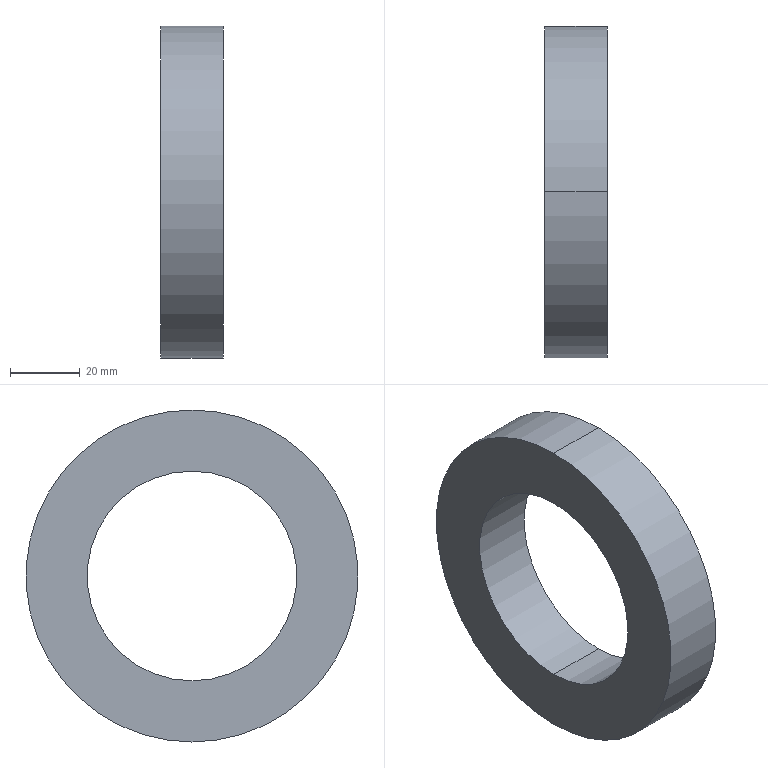Component | SolidWorks | 6012-1 | 1 solid | 6 faces | box 18 x 95 x 95 mm | volume 76694 mm3 | cylinder 4 | plane 2 | commonest cylinder face diameters 60 x2 95 x2
build123d program:
from build123d import *

# Parameters (mm, degrees)
SKETCH1_R           = 47.5
SKETCH1_R_2         = 30
BOSS_EXTRUDE1_DEPTH = 9


with BuildPart() as part:
    # Sketch1 → Boss-Extrude1 (new, symmetric)
    with BuildSketch(Plane(origin=(0, 0, 0), x_dir=(0, 0, -1), z_dir=(1, 0, 0))):
        Circle(SKETCH1_R)
        Circle(SKETCH1_R_2, mode=Mode.SUBTRACT)
    extrude(amount=BOSS_EXTRUDE1_DEPTH, both=True)


solid = part.part

# Placed as in the assembly
solid = solid.moved(Location((572.303, 34.532, 0), (0, 0, 0)))
STEP:
#1=COLOUR_RGB('',0.7922,0.8196,0.9333);
#2=FILL_AREA_STYLE_COLOUR('',#1);
#3=FILL_AREA_STYLE('',(#2));
#4=SURFACE_STYLE_FILL_AREA(#3);
#5=SURFACE_SIDE_STYLE('',(#4));
#6=SURFACE_STYLE_USAGE(.BOTH.,#5);
#7=PRESENTATION_STYLE_ASSIGNMENT((#6));
#8=CARTESIAN_POINT('',(22.886,1.36,1.181));
#9=VERTEX_POINT('',#8);
#10=CARTESIAN_POINT('',(22.886,1.36,-1.181));
#11=VERTEX_POINT('',#10);
#12=CARTESIAN_POINT('',(22.886,1.36,0.));
#13=DIRECTION('',(1.,0.,0.));
#14=DIRECTION('',(0.,0.,-1.));
#15=AXIS2_PLACEMENT_3D('',#12,#13,#14);
#16=CIRCLE('',#15,1.181);
#17=EDGE_CURVE('',#9,#11,#16,.T.);
#18=ORIENTED_EDGE('',*,*,#17,.T.);
#19=CARTESIAN_POINT('',(22.177,1.36,-1.181));
#20=VERTEX_POINT('',#19);
#21=CARTESIAN_POINT('',(22.886,1.36,-1.181));
#22=DIRECTION('',(-1.,0.,0.));
#23=VECTOR('',#22,39.37);
#24=LINE('',#21,#23);
#25=EDGE_CURVE('',#11,#20,#24,.T.);
#26=ORIENTED_EDGE('',*,*,#25,.T.);
#27=CARTESIAN_POINT('',(22.177,1.36,1.181));
#28=VERTEX_POINT('',#27);
#29=CARTESIAN_POINT('',(22.177,1.36,0.));
#30=DIRECTION('',(1.,0.,0.));
#31=DIRECTION('',(0.,0.,-1.));
#32=AXIS2_PLACEMENT_3D('',#29,#30,#31);
#33=CIRCLE('',#32,1.181);
#34=EDGE_CURVE('',#28,#20,#33,.T.);
#35=ORIENTED_EDGE('',*,*,#34,.F.);
#36=CARTESIAN_POINT('',(22.886,1.36,1.181));
#37=DIRECTION('',(-1.,0.,0.));
#38=VECTOR('',#37,39.37);
#39=LINE('',#36,#38);
#40=EDGE_CURVE('',#9,#28,#39,.T.);
#41=ORIENTED_EDGE('',*,*,#40,.F.);
#42=EDGE_LOOP('',(#18,#26,#35,#41));
#43=FACE_OUTER_BOUND('',#42,.T.);
#44=CARTESIAN_POINT('',(22.886,1.36,0.));
#45=DIRECTION('',(-1.,0.,0.));
#46=DIRECTION('',(0.,0.,1.));
#47=AXIS2_PLACEMENT_3D('',#44,#45,#46);
#48=CYLINDRICAL_SURFACE('',#47,1.181);
#49=ADVANCED_FACE('',(#43),#48,.F.);
#50=CARTESIAN_POINT('',(22.886,1.36,-1.87));
#51=VERTEX_POINT('',#50);
#52=CARTESIAN_POINT('',(22.886,1.36,1.87));
#53=VERTEX_POINT('',#52);
#54=CARTESIAN_POINT('',(22.886,1.36,0.));
#55=DIRECTION('',(1.,0.,0.));
#56=DIRECTION('',(0.,0.,-1.));
#57=AXIS2_PLACEMENT_3D('',#54,#55,#56);
#58=CIRCLE('',#57,1.87);
#59=EDGE_CURVE('',#51,#53,#58,.T.);
#60=ORIENTED_EDGE('',*,*,#59,.F.);
#61=CARTESIAN_POINT('',(22.177,1.36,-1.87));
#62=VERTEX_POINT('',#61);
#63=CARTESIAN_POINT('',(22.886,1.36,-1.87));
#64=DIRECTION('',(-1.,0.,0.));
#65=VECTOR('',#64,39.37);
#66=LINE('',#63,#65);
#67=EDGE_CURVE('',#51,#62,#66,.T.);
#68=ORIENTED_EDGE('',*,*,#67,.T.);
#69=CARTESIAN_POINT('',(22.177,1.36,1.87));
#70=VERTEX_POINT('',#69);
#71=CARTESIAN_POINT('',(22.177,1.36,0.));
#72=DIRECTION('',(1.,0.,0.));
#73=DIRECTION('',(0.,0.,-1.));
#74=AXIS2_PLACEMENT_3D('',#71,#72,#73);
#75=CIRCLE('',#74,1.87);
#76=EDGE_CURVE('',#62,#70,#75,.T.);
#77=ORIENTED_EDGE('',*,*,#76,.T.);
#78=CARTESIAN_POINT('',(22.886,1.36,1.87));
#79=DIRECTION('',(-1.,0.,0.));
#80=VECTOR('',#79,39.37);
#81=LINE('',#78,#80);
#82=EDGE_CURVE('',#53,#70,#81,.T.);
#83=ORIENTED_EDGE('',*,*,#82,.F.);
#84=EDGE_LOOP('',(#60,#68,#77,#83));
#85=FACE_OUTER_BOUND('',#84,.T.);
#86=CARTESIAN_POINT('',(22.886,1.36,0.));
#87=DIRECTION('',(-1.,0.,0.));
#88=DIRECTION('',(0.,0.,1.));
#89=AXIS2_PLACEMENT_3D('',#86,#87,#88);
#90=CYLINDRICAL_SURFACE('',#89,1.87);
#91=ADVANCED_FACE('',(#85),#90,.T.);
#92=CARTESIAN_POINT('',(22.886,1.36,0.));
#93=DIRECTION('',(1.,0.,0.));
#94=DIRECTION('',(0.,0.,-1.));
#95=AXIS2_PLACEMENT_3D('',#92,#93,#94);
#96=CIRCLE('',#95,1.87);
#97=EDGE_CURVE('',#53,#51,#96,.T.);
#98=ORIENTED_EDGE('',*,*,#97,.T.);
#99=ORIENTED_EDGE('',*,*,#59,.T.);
#100=EDGE_LOOP('',(#98,#99));
#101=FACE_OUTER_BOUND('',#100,.T.);
#102=ORIENTED_EDGE('',*,*,#17,.F.);
#103=CARTESIAN_POINT('',(22.886,1.36,0.));
#104=DIRECTION('',(1.,0.,0.));
#105=DIRECTION('',(0.,0.,-1.));
#106=AXIS2_PLACEMENT_3D('',#103,#104,#105);
#107=CIRCLE('',#106,1.181);
#108=EDGE_CURVE('',#11,#9,#107,.T.);
#109=ORIENTED_EDGE('',*,*,#108,.F.);
#110=EDGE_LOOP('',(#102,#109));
#111=FACE_BOUND('',#110,.T.);
#112=CARTESIAN_POINT('',(22.886,1.36,0.));
#113=DIRECTION('',(1.,0.,0.));
#114=DIRECTION('',(0.,0.,-1.));
#115=AXIS2_PLACEMENT_3D('',#112,#113,#114);
#116=PLANE('',#115);
#117=ADVANCED_FACE('',(#101,#111),#116,.T.);
#118=CARTESIAN_POINT('',(22.177,1.36,0.));
#119=DIRECTION('',(1.,0.,0.));
#120=DIRECTION('',(0.,0.,-1.));
#121=AXIS2_PLACEMENT_3D('',#118,#119,#120);
#122=CIRCLE('',#121,1.87);
#123=EDGE_CURVE('',#70,#62,#122,.T.);
#124=ORIENTED_EDGE('',*,*,#123,.F.);
#125=ORIENTED_EDGE('',*,*,#76,.F.);
#126=EDGE_LOOP('',(#124,#125));
#127=FACE_OUTER_BOUND('',#126,.T.);
#128=ORIENTED_EDGE('',*,*,#34,.T.);
#129=CARTESIAN_POINT('',(22.177,1.36,0.));
#130=DIRECTION('',(1.,0.,0.));
#131=DIRECTION('',(0.,0.,-1.));
#132=AXIS2_PLACEMENT_3D('',#129,#130,#131);
#133=CIRCLE('',#132,1.181);
#134=EDGE_CURVE('',#20,#28,#133,.T.);
#135=ORIENTED_EDGE('',*,*,#134,.T.);
#136=EDGE_LOOP('',(#128,#135));
#137=FACE_BOUND('',#136,.T.);
#138=CARTESIAN_POINT('',(22.177,1.36,0.));
#139=DIRECTION('',(1.,0.,0.));
#140=DIRECTION('',(0.,0.,-1.));
#141=AXIS2_PLACEMENT_3D('',#138,#139,#140);
#142=PLANE('',#141);
#143=ADVANCED_FACE('',(#127,#137),#142,.F.);
#144=ORIENTED_EDGE('',*,*,#67,.F.);
#145=ORIENTED_EDGE('',*,*,#97,.F.);
#146=ORIENTED_EDGE('',*,*,#82,.T.);
#147=ORIENTED_EDGE('',*,*,#123,.T.);
#148=EDGE_LOOP('',(#144,#145,#146,#147));
#149=FACE_OUTER_BOUND('',#148,.T.);
#150=CARTESIAN_POINT('',(22.886,1.36,0.));
#151=DIRECTION('',(-1.,0.,0.));
#152=DIRECTION('',(0.,0.,1.));
#153=AXIS2_PLACEMENT_3D('',#150,#151,#152);
#154=CYLINDRICAL_SURFACE('',#153,1.87);
#155=ADVANCED_FACE('',(#149),#154,.T.);
#156=ORIENTED_EDGE('',*,*,#25,.F.);
#157=ORIENTED_EDGE('',*,*,#108,.T.);
#158=ORIENTED_EDGE('',*,*,#40,.T.);
#159=ORIENTED_EDGE('',*,*,#134,.F.);
#160=EDGE_LOOP('',(#156,#157,#158,#159));
#161=FACE_OUTER_BOUND('',#160,.T.);
#162=CARTESIAN_POINT('',(22.886,1.36,0.));
#163=DIRECTION('',(-1.,0.,0.));
#164=DIRECTION('',(0.,0.,1.));
#165=AXIS2_PLACEMENT_3D('',#162,#163,#164);
#166=CYLINDRICAL_SURFACE('',#165,1.181);
#167=ADVANCED_FACE('',(#161),#166,.F.);
#168=CLOSED_SHELL('',(#49,#91,#117,#143,#155,#167));
#169=MANIFOLD_SOLID_BREP('',#168);
#170=STYLED_ITEM('',(#7),#169);
#171=PRESENTATION_LAYER_ASSIGNMENT('','',(#170));
#172=CARTESIAN_POINT('',(0.,0.,0.));
#173=DIRECTION('',(0.,0.,1.));
#174=DIRECTION('',(1.,0.,0.));
#175=AXIS2_PLACEMENT_3D('',#172,#173,#174);
#176=(LENGTH_UNIT()NAMED_UNIT(*)SI_UNIT($,.METRE.));
#177=LENGTH_MEASURE_WITH_UNIT(LENGTH_MEASURE(0.0254),#176);
#178=DIMENSIONAL_EXPONENTS(1.,0.,0.,0.,0.,0.,0.);
#179=(CONVERSION_BASED_UNIT('',#177)LENGTH_UNIT()NAMED_UNIT(#178));
#180=UNCERTAINTY_MEASURE_WITH_UNIT(LENGTH_MEASURE(0.00001),#179,'','');
#181=(NAMED_UNIT(*)PLANE_ANGLE_UNIT()SI_UNIT($,.RADIAN.));
#182=(NAMED_UNIT(*)SI_UNIT($,.STERADIAN.)SOLID_ANGLE_UNIT());
#183=(GEOMETRIC_REPRESENTATION_CONTEXT(3)GLOBAL_UNCERTAINTY_ASSIGNED_CONTEXT((#180))GLOBAL_UNIT_ASSIGNED_CONTEXT((#179,#181,#182))REPRESENTATION_CONTEXT('',''));
#184=ADVANCED_BREP_SHAPE_REPRESENTATION('',(#169,#175),#183);
#185=(LENGTH_UNIT()NAMED_UNIT(*)SI_UNIT($,.METRE.));
#186=LENGTH_MEASURE_WITH_UNIT(LENGTH_MEASURE(0.0254),#185);
#187=DIMENSIONAL_EXPONENTS(1.,0.,0.,0.,0.,0.,0.);
#188=(CONVERSION_BASED_UNIT('',#186)LENGTH_UNIT()NAMED_UNIT(#187));
#189=UNCERTAINTY_MEASURE_WITH_UNIT(LENGTH_MEASURE(0.00001),#188,'','');
#190=(NAMED_UNIT(*)PLANE_ANGLE_UNIT()SI_UNIT($,.RADIAN.));
#191=(NAMED_UNIT(*)SI_UNIT($,.STERADIAN.)SOLID_ANGLE_UNIT());
#192=(GEOMETRIC_REPRESENTATION_CONTEXT(3)GLOBAL_UNCERTAINTY_ASSIGNED_CONTEXT((#189))GLOBAL_UNIT_ASSIGNED_CONTEXT((#188,#190,#191))REPRESENTATION_CONTEXT('',''));
#193=MECHANICAL_DESIGN_GEOMETRIC_PRESENTATION_REPRESENTATION('',(#170),#192);